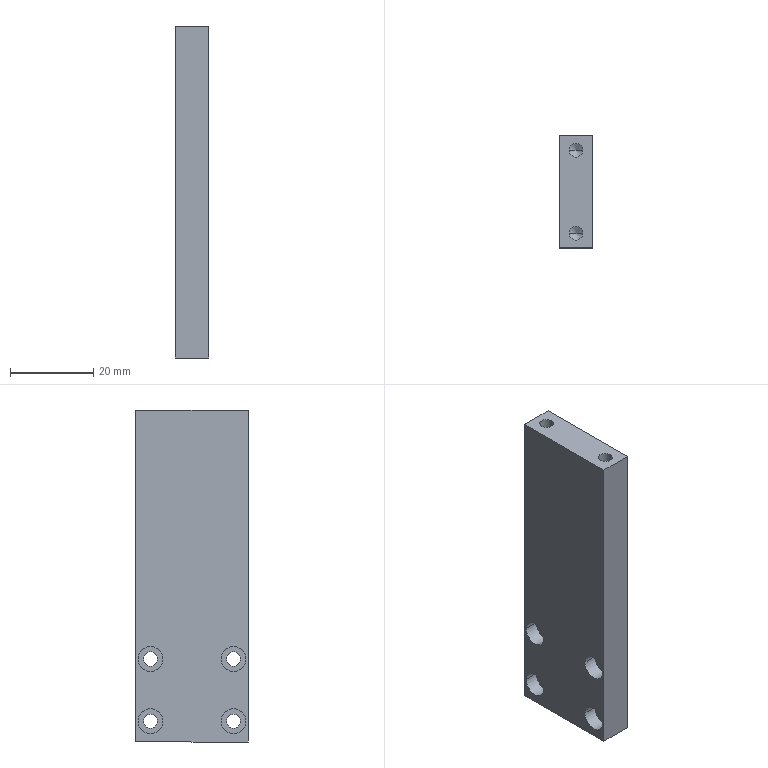Component | SolidWorks | JQ-2-0-004-2 | 1 solid | 34 faces | box 8 x 27 x 80 mm | volume 16526 mm3 | cylinder 20 | plane 10 | cone 4 | commonest cylinder face diameters 6 x8 3.4 x8 3.3 x4
build123d program:
from build123d import *

# Parameters (mm, degrees)
SKETCH1_W                                            = 27
SKETCH1_H                                            = 80
BOSS_EXTRUDE1_DEPTH                                  = 8
HOLE_SIZE_ACCORDING_TO_TYPE_1_OF_HEX_SOC_D           = 3.4
HOLE_SIZE_ACCORDING_TO_TYPE_1_OF_HEX_SOC_CBORE_D     = 6
HOLE_SIZE_ACCORDING_TO_TYPE_1_OF_HEX_SOC_CBORE_DEPTH = 3.4
M4_TAPPED_HOLE1_D                                    = 3.3
M4_TAPPED_HOLE1_DEPTH                                = 11.5
M4_TAPPED_HOLE1_TIP                                  = 0.9914


with BuildPart() as part:
    # Sketch1 → Boss-Extrude1 (new body)
    with BuildSketch(Plane.XY):
        with Locations((13.5, 40)):
            Rectangle(SKETCH1_W, SKETCH1_H)
    extrude(amount=BOSS_EXTRUDE1_DEPTH)

    # Hole Size according to type 1 of hex soc (through all)
    with Locations(Plane.XY.offset(8)):
        with Locations((3.5, 5), (23.5, 5), (3.5, 20), (23.5, 20)):
            CounterBoreHole(HOLE_SIZE_ACCORDING_TO_TYPE_1_OF_HEX_SOC_D / 2, HOLE_SIZE_ACCORDING_TO_TYPE_1_OF_HEX_SOC_CBORE_D / 2, HOLE_SIZE_ACCORDING_TO_TYPE_1_OF_HEX_SOC_CBORE_DEPTH)

    # M4 Tapped Hole1
    with Locations(Plane(origin=(0, 80, 0), x_dir=(-1, 0, 0), z_dir=(0, 1, 0))):
        with Locations((-23.5, 4), (-3.5, 4)):
            Hole(M4_TAPPED_HOLE1_D / 2, depth=M4_TAPPED_HOLE1_DEPTH)
            with Locations((0, 0, -(M4_TAPPED_HOLE1_DEPTH + M4_TAPPED_HOLE1_TIP / 2))):  # 118° drill point
                Cone(0, M4_TAPPED_HOLE1_D / 2, M4_TAPPED_HOLE1_TIP, mode=Mode.SUBTRACT)


solid = part.part

# Placed as in the assembly
solid = solid.moved(Location((-355.058, 42.839, 19.131), (90, -90, 0)))
STEP:
#1=COLOUR_RGB('',0.7922,0.8196,0.9333);
#2=FILL_AREA_STYLE_COLOUR('',#1);
#3=FILL_AREA_STYLE('',(#2));
#4=SURFACE_STYLE_FILL_AREA(#3);
#5=SURFACE_SIDE_STYLE('',(#4));
#6=SURFACE_STYLE_USAGE(.BOTH.,#5);
#7=PRESENTATION_STYLE_ASSIGNMENT((#6));
#8=CARTESIAN_POINT('',(-14.071,0.7614,3.45));
#9=VERTEX_POINT('',#8);
#10=CARTESIAN_POINT('',(-14.201,0.7614,3.45));
#11=VERTEX_POINT('',#10);
#12=CARTESIAN_POINT('',(-14.136,0.7614,3.45));
#13=DIRECTION('',(-0.,-0.,1.));
#14=DIRECTION('',(-1.,0.,0.));
#15=AXIS2_PLACEMENT_3D('',#12,#13,#14);
#16=CIRCLE('',#15,0.06496);
#17=EDGE_CURVE('',#9,#11,#16,.T.);
#18=ORIENTED_EDGE('',*,*,#17,.F.);
#19=CARTESIAN_POINT('',(-14.071,0.7614,3.903));
#20=VERTEX_POINT('',#19);
#21=CARTESIAN_POINT('',(-14.071,0.7614,3.903));
#22=DIRECTION('',(-0.,-0.,1.));
#23=VECTOR('',#22,39.37);
#24=LINE('',#21,#23);
#25=EDGE_CURVE('',#9,#20,#24,.T.);
#26=ORIENTED_EDGE('',*,*,#25,.T.);
#27=CARTESIAN_POINT('',(-14.201,0.7614,3.903));
#28=VERTEX_POINT('',#27);
#29=CARTESIAN_POINT('',(-14.136,0.7614,3.903));
#30=DIRECTION('',(-0.,-0.,1.));
#31=DIRECTION('',(-1.,0.,0.));
#32=AXIS2_PLACEMENT_3D('',#29,#30,#31);
#33=CIRCLE('',#32,0.06496);
#34=EDGE_CURVE('',#20,#28,#33,.T.);
#35=ORIENTED_EDGE('',*,*,#34,.T.);
#36=CARTESIAN_POINT('',(-14.201,0.7614,3.903));
#37=DIRECTION('',(-0.,-0.,1.));
#38=VECTOR('',#37,39.37);
#39=LINE('',#36,#38);
#40=EDGE_CURVE('',#11,#28,#39,.T.);
#41=ORIENTED_EDGE('',*,*,#40,.F.);
#42=EDGE_LOOP('',(#18,#26,#35,#41));
#43=FACE_OUTER_BOUND('',#42,.T.);
#44=CARTESIAN_POINT('',(-14.136,0.7614,3.903));
#45=DIRECTION('',(-0.,-0.,1.));
#46=DIRECTION('',(-1.,0.,0.));
#47=AXIS2_PLACEMENT_3D('',#44,#45,#46);
#48=CYLINDRICAL_SURFACE('',#47,0.06496);
#49=ADVANCED_FACE('',(#43),#48,.F.);
#50=CARTESIAN_POINT('',(-14.136,0.7614,3.411));
#51=VERTEX_POINT('',#50);
#52=CARTESIAN_POINT('',(-14.201,0.7614,3.45));
#53=DIRECTION('',(-0.8572,0.,0.515));
#54=VECTOR('',#53,39.37);
#55=LINE('',#52,#54);
#56=EDGE_CURVE('',#51,#11,#55,.T.);
#57=ORIENTED_EDGE('',*,*,#56,.F.);
#58=CARTESIAN_POINT('',(-14.071,0.7614,3.45));
#59=DIRECTION('',(0.8572,-0.,0.515));
#60=VECTOR('',#59,39.37);
#61=LINE('',#58,#60);
#62=EDGE_CURVE('',#51,#9,#61,.T.);
#63=ORIENTED_EDGE('',*,*,#62,.T.);
#64=ORIENTED_EDGE('',*,*,#17,.T.);
#65=EDGE_LOOP('',(#57,#63,#64));
#66=FACE_OUTER_BOUND('',#65,.T.);
#67=CARTESIAN_POINT('',(-14.136,0.7614,3.45));
#68=DIRECTION('',(-0.,-0.,1.));
#69=DIRECTION('',(-1.,0.,0.));
#70=AXIS2_PLACEMENT_3D('',#67,#68,#69);
#71=CONICAL_SURFACE('',#70,0.06496,1.03);
#72=ADVANCED_FACE('',(#66),#71,.F.);
#73=CARTESIAN_POINT('',(-14.071,1.549,3.45));
#74=VERTEX_POINT('',#73);
#75=CARTESIAN_POINT('',(-14.201,1.549,3.45));
#76=VERTEX_POINT('',#75);
#77=CARTESIAN_POINT('',(-14.136,1.549,3.45));
#78=DIRECTION('',(-0.,-0.,1.));
#79=DIRECTION('',(-1.,0.,0.));
#80=AXIS2_PLACEMENT_3D('',#77,#78,#79);
#81=CIRCLE('',#80,0.06496);
#82=EDGE_CURVE('',#74,#76,#81,.T.);
#83=ORIENTED_EDGE('',*,*,#82,.F.);
#84=CARTESIAN_POINT('',(-14.071,1.549,3.903));
#85=VERTEX_POINT('',#84);
#86=CARTESIAN_POINT('',(-14.071,1.549,3.903));
#87=DIRECTION('',(-0.,-0.,1.));
#88=VECTOR('',#87,39.37);
#89=LINE('',#86,#88);
#90=EDGE_CURVE('',#74,#85,#89,.T.);
#91=ORIENTED_EDGE('',*,*,#90,.T.);
#92=CARTESIAN_POINT('',(-14.201,1.549,3.903));
#93=VERTEX_POINT('',#92);
#94=CARTESIAN_POINT('',(-14.136,1.549,3.903));
#95=DIRECTION('',(-0.,-0.,1.));
#96=DIRECTION('',(-1.,0.,0.));
#97=AXIS2_PLACEMENT_3D('',#94,#95,#96);
#98=CIRCLE('',#97,0.06496);
#99=EDGE_CURVE('',#85,#93,#98,.T.);
#100=ORIENTED_EDGE('',*,*,#99,.T.);
#101=CARTESIAN_POINT('',(-14.201,1.549,3.903));
#102=DIRECTION('',(-0.,-0.,1.));
#103=VECTOR('',#102,39.37);
#104=LINE('',#101,#103);
#105=EDGE_CURVE('',#76,#93,#104,.T.);
#106=ORIENTED_EDGE('',*,*,#105,.F.);
#107=EDGE_LOOP('',(#83,#91,#100,#106));
#108=FACE_OUTER_BOUND('',#107,.T.);
#109=CARTESIAN_POINT('',(-14.136,1.549,3.903));
#110=DIRECTION('',(-0.,-0.,1.));
#111=DIRECTION('',(-1.,0.,0.));
#112=AXIS2_PLACEMENT_3D('',#109,#110,#111);
#113=CYLINDRICAL_SURFACE('',#112,0.06496);
#114=ADVANCED_FACE('',(#108),#113,.F.);
#115=CARTESIAN_POINT('',(-14.136,1.549,3.411));
#116=VERTEX_POINT('',#115);
#117=CARTESIAN_POINT('',(-14.201,1.549,3.45));
#118=DIRECTION('',(-0.8572,0.,0.515));
#119=VECTOR('',#118,39.37);
#120=LINE('',#117,#119);
#121=EDGE_CURVE('',#116,#76,#120,.T.);
#122=ORIENTED_EDGE('',*,*,#121,.F.);
#123=CARTESIAN_POINT('',(-14.071,1.549,3.45));
#124=DIRECTION('',(0.8572,-0.,0.515));
#125=VECTOR('',#124,39.37);
#126=LINE('',#123,#125);
#127=EDGE_CURVE('',#116,#74,#126,.T.);
#128=ORIENTED_EDGE('',*,*,#127,.T.);
#129=ORIENTED_EDGE('',*,*,#82,.T.);
#130=EDGE_LOOP('',(#122,#128,#129));
#131=FACE_OUTER_BOUND('',#130,.T.);
#132=CARTESIAN_POINT('',(-14.136,1.549,3.45));
#133=DIRECTION('',(-0.,-0.,1.));
#134=DIRECTION('',(-1.,0.,0.));
#135=AXIS2_PLACEMENT_3D('',#132,#133,#134);
#136=CONICAL_SURFACE('',#135,0.06496,1.03);
#137=ADVANCED_FACE('',(#131),#136,.F.);
#138=CARTESIAN_POINT('',(-14.16,1.667,0.95));
#139=VERTEX_POINT('',#138);
#140=CARTESIAN_POINT('',(-14.16,1.431,0.95));
#141=VERTEX_POINT('',#140);
#142=CARTESIAN_POINT('',(-14.16,1.549,0.95));
#143=DIRECTION('',(-1.,0.,-0.));
#144=DIRECTION('',(0.,-1.,0.));
#145=AXIS2_PLACEMENT_3D('',#142,#143,#144);
#146=CIRCLE('',#145,0.1181);
#147=EDGE_CURVE('',#139,#141,#146,.T.);
#148=ORIENTED_EDGE('',*,*,#147,.F.);
#149=CARTESIAN_POINT('',(-14.294,1.667,0.95));
#150=VERTEX_POINT('',#149);
#151=CARTESIAN_POINT('',(-14.294,1.667,0.95));
#152=DIRECTION('',(-1.,0.,-0.));
#153=VECTOR('',#152,39.37);
#154=LINE('',#151,#153);
#155=EDGE_CURVE('',#139,#150,#154,.T.);
#156=ORIENTED_EDGE('',*,*,#155,.T.);
#157=CARTESIAN_POINT('',(-14.294,1.431,0.95));
#158=VERTEX_POINT('',#157);
#159=CARTESIAN_POINT('',(-14.294,1.549,0.95));
#160=DIRECTION('',(-1.,0.,-0.));
#161=DIRECTION('',(0.,-1.,0.));
#162=AXIS2_PLACEMENT_3D('',#159,#160,#161);
#163=CIRCLE('',#162,0.1181);
#164=EDGE_CURVE('',#150,#158,#163,.T.);
#165=ORIENTED_EDGE('',*,*,#164,.T.);
#166=CARTESIAN_POINT('',(-14.294,1.431,0.95));
#167=DIRECTION('',(-1.,0.,-0.));
#168=VECTOR('',#167,39.37);
#169=LINE('',#166,#168);
#170=EDGE_CURVE('',#141,#158,#169,.T.);
#171=ORIENTED_EDGE('',*,*,#170,.F.);
#172=EDGE_LOOP('',(#148,#156,#165,#171));
#173=FACE_OUTER_BOUND('',#172,.T.);
#174=CARTESIAN_POINT('',(-14.294,1.549,0.95));
#175=DIRECTION('',(-1.,0.,-0.));
#176=DIRECTION('',(0.,-1.,0.));
#177=AXIS2_PLACEMENT_3D('',#174,#175,#176);
#178=CYLINDRICAL_SURFACE('',#177,0.1181);
#179=ADVANCED_FACE('',(#173),#178,.F.);
#180=CARTESIAN_POINT('',(-13.979,1.616,0.95));
#181=VERTEX_POINT('',#180);
#182=CARTESIAN_POINT('',(-13.979,1.482,0.95));
#183=VERTEX_POINT('',#182);
#184=CARTESIAN_POINT('',(-13.979,1.549,0.95));
#185=DIRECTION('',(-1.,0.,-0.));
#186=DIRECTION('',(0.,-1.,0.));
#187=AXIS2_PLACEMENT_3D('',#184,#185,#186);
#188=CIRCLE('',#187,0.06693);
#189=EDGE_CURVE('',#181,#183,#188,.T.);
#190=ORIENTED_EDGE('',*,*,#189,.F.);
#191=CARTESIAN_POINT('',(-14.16,1.616,0.95));
#192=VERTEX_POINT('',#191);
#193=CARTESIAN_POINT('',(-14.294,1.616,0.95));
#194=DIRECTION('',(-1.,0.,-0.));
#195=VECTOR('',#194,39.37);
#196=LINE('',#193,#195);
#197=EDGE_CURVE('',#181,#192,#196,.T.);
#198=ORIENTED_EDGE('',*,*,#197,.T.);
#199=CARTESIAN_POINT('',(-14.16,1.482,0.95));
#200=VERTEX_POINT('',#199);
#201=CARTESIAN_POINT('',(-14.16,1.549,0.95));
#202=DIRECTION('',(-1.,0.,-0.));
#203=DIRECTION('',(0.,-1.,0.));
#204=AXIS2_PLACEMENT_3D('',#201,#202,#203);
#205=CIRCLE('',#204,0.06693);
#206=EDGE_CURVE('',#192,#200,#205,.T.);
#207=ORIENTED_EDGE('',*,*,#206,.T.);
#208=CARTESIAN_POINT('',(-14.294,1.482,0.95));
#209=DIRECTION('',(-1.,0.,-0.));
#210=VECTOR('',#209,39.37);
#211=LINE('',#208,#210);
#212=EDGE_CURVE('',#183,#200,#211,.T.);
#213=ORIENTED_EDGE('',*,*,#212,.F.);
#214=EDGE_LOOP('',(#190,#198,#207,#213));
#215=FACE_OUTER_BOUND('',#214,.T.);
#216=CARTESIAN_POINT('',(-14.294,1.549,0.95));
#217=DIRECTION('',(-1.,0.,-0.));
#218=DIRECTION('',(0.,-1.,0.));
#219=AXIS2_PLACEMENT_3D('',#216,#217,#218);
#220=CYLINDRICAL_SURFACE('',#219,0.06693);
#221=ADVANCED_FACE('',(#215),#220,.F.);
#222=CARTESIAN_POINT('',(-14.16,0.8795,0.95));
#223=VERTEX_POINT('',#222);
#224=CARTESIAN_POINT('',(-14.16,0.6433,0.95));
#225=VERTEX_POINT('',#224);
#226=CARTESIAN_POINT('',(-14.16,0.7614,0.95));
#227=DIRECTION('',(-1.,0.,-0.));
#228=DIRECTION('',(0.,-1.,0.));
#229=AXIS2_PLACEMENT_3D('',#226,#227,#228);
#230=CIRCLE('',#229,0.1181);
#231=EDGE_CURVE('',#223,#225,#230,.T.);
#232=ORIENTED_EDGE('',*,*,#231,.F.);
#233=CARTESIAN_POINT('',(-14.294,0.8795,0.95));
#234=VERTEX_POINT('',#233);
#235=CARTESIAN_POINT('',(-14.294,0.8795,0.95));
#236=DIRECTION('',(-1.,0.,-0.));
#237=VECTOR('',#236,39.37);
#238=LINE('',#235,#237);
#239=EDGE_CURVE('',#223,#234,#238,.T.);
#240=ORIENTED_EDGE('',*,*,#239,.T.);
#241=CARTESIAN_POINT('',(-14.294,0.6433,0.95));
#242=VERTEX_POINT('',#241);
#243=CARTESIAN_POINT('',(-14.294,0.7614,0.95));
#244=DIRECTION('',(-1.,0.,-0.));
#245=DIRECTION('',(0.,-1.,0.));
#246=AXIS2_PLACEMENT_3D('',#243,#244,#245);
#247=CIRCLE('',#246,0.1181);
#248=EDGE_CURVE('',#234,#242,#247,.T.);
#249=ORIENTED_EDGE('',*,*,#248,.T.);
#250=CARTESIAN_POINT('',(-14.294,0.6433,0.95));
#251=DIRECTION('',(-1.,0.,-0.));
#252=VECTOR('',#251,39.37);
#253=LINE('',#250,#252);
#254=EDGE_CURVE('',#225,#242,#253,.T.);
#255=ORIENTED_EDGE('',*,*,#254,.F.);
#256=EDGE_LOOP('',(#232,#240,#249,#255));
#257=FACE_OUTER_BOUND('',#256,.T.);
#258=CARTESIAN_POINT('',(-14.294,0.7614,0.95));
#259=DIRECTION('',(-1.,0.,-0.));
#260=DIRECTION('',(0.,-1.,0.));
#261=AXIS2_PLACEMENT_3D('',#258,#259,#260);
#262=CYLINDRICAL_SURFACE('',#261,0.1181);
#263=ADVANCED_FACE('',(#257),#262,.F.);
#264=CARTESIAN_POINT('',(-13.979,0.8283,0.95));
#265=VERTEX_POINT('',#264);
#266=CARTESIAN_POINT('',(-13.979,0.6945,0.95));
#267=VERTEX_POINT('',#266);
#268=CARTESIAN_POINT('',(-13.979,0.7614,0.95));
#269=DIRECTION('',(-1.,0.,-0.));
#270=DIRECTION('',(0.,-1.,0.));
#271=AXIS2_PLACEMENT_3D('',#268,#269,#270);
#272=CIRCLE('',#271,0.06693);
#273=EDGE_CURVE('',#265,#267,#272,.T.);
#274=ORIENTED_EDGE('',*,*,#273,.F.);
#275=CARTESIAN_POINT('',(-14.16,0.8283,0.95));
#276=VERTEX_POINT('',#275);
#277=CARTESIAN_POINT('',(-14.294,0.8283,0.95));
#278=DIRECTION('',(-1.,0.,-0.));
#279=VECTOR('',#278,39.37);
#280=LINE('',#277,#279);
#281=EDGE_CURVE('',#265,#276,#280,.T.);
#282=ORIENTED_EDGE('',*,*,#281,.T.);
#283=CARTESIAN_POINT('',(-14.16,0.6945,0.95));
#284=VERTEX_POINT('',#283);
#285=CARTESIAN_POINT('',(-14.16,0.7614,0.95));
#286=DIRECTION('',(-1.,0.,-0.));
#287=DIRECTION('',(0.,-1.,0.));
#288=AXIS2_PLACEMENT_3D('',#285,#286,#287);
#289=CIRCLE('',#288,0.06693);
#290=EDGE_CURVE('',#276,#284,#289,.T.);
#291=ORIENTED_EDGE('',*,*,#290,.T.);
#292=CARTESIAN_POINT('',(-14.294,0.6945,0.95));
#293=DIRECTION('',(-1.,0.,-0.));
#294=VECTOR('',#293,39.37);
#295=LINE('',#292,#294);
#296=EDGE_CURVE('',#267,#284,#295,.T.);
#297=ORIENTED_EDGE('',*,*,#296,.F.);
#298=EDGE_LOOP('',(#274,#282,#291,#297));
#299=FACE_OUTER_BOUND('',#298,.T.);
#300=CARTESIAN_POINT('',(-14.294,0.7614,0.95));
#301=DIRECTION('',(-1.,0.,-0.));
#302=DIRECTION('',(0.,-1.,0.));
#303=AXIS2_PLACEMENT_3D('',#300,#301,#302);
#304=CYLINDRICAL_SURFACE('',#303,0.06693);
#305=ADVANCED_FACE('',(#299),#304,.F.);
#306=CARTESIAN_POINT('',(-14.16,1.667,1.541));
#307=VERTEX_POINT('',#306);
#308=CARTESIAN_POINT('',(-14.16,1.431,1.541));
#309=VERTEX_POINT('',#308);
#310=CARTESIAN_POINT('',(-14.16,1.549,1.541));
#311=DIRECTION('',(-1.,0.,-0.));
#312=DIRECTION('',(0.,-1.,0.));
#313=AXIS2_PLACEMENT_3D('',#310,#311,#312);
#314=CIRCLE('',#313,0.1181);
#315=EDGE_CURVE('',#307,#309,#314,.T.);
#316=ORIENTED_EDGE('',*,*,#315,.F.);
#317=CARTESIAN_POINT('',(-14.294,1.667,1.541));
#318=VERTEX_POINT('',#317);
#319=CARTESIAN_POINT('',(-14.294,1.667,1.541));
#320=DIRECTION('',(-1.,0.,-0.));
#321=VECTOR('',#320,39.37);
#322=LINE('',#319,#321);
#323=EDGE_CURVE('',#307,#318,#322,.T.);
#324=ORIENTED_EDGE('',*,*,#323,.T.);
#325=CARTESIAN_POINT('',(-14.294,1.431,1.541));
#326=VERTEX_POINT('',#325);
#327=CARTESIAN_POINT('',(-14.294,1.549,1.541));
#328=DIRECTION('',(-1.,0.,-0.));
#329=DIRECTION('',(0.,-1.,0.));
#330=AXIS2_PLACEMENT_3D('',#327,#328,#329);
#331=CIRCLE('',#330,0.1181);
#332=EDGE_CURVE('',#318,#326,#331,.T.);
#333=ORIENTED_EDGE('',*,*,#332,.T.);
#334=CARTESIAN_POINT('',(-14.294,1.431,1.541));
#335=DIRECTION('',(-1.,0.,-0.));
#336=VECTOR('',#335,39.37);
#337=LINE('',#334,#336);
#338=EDGE_CURVE('',#309,#326,#337,.T.);
#339=ORIENTED_EDGE('',*,*,#338,.F.);
#340=EDGE_LOOP('',(#316,#324,#333,#339));
#341=FACE_OUTER_BOUND('',#340,.T.);
#342=CARTESIAN_POINT('',(-14.294,1.549,1.541));
#343=DIRECTION('',(-1.,0.,-0.));
#344=DIRECTION('',(0.,-1.,0.));
#345=AXIS2_PLACEMENT_3D('',#342,#343,#344);
#346=CYLINDRICAL_SURFACE('',#345,0.1181);
#347=ADVANCED_FACE('',(#341),#346,.F.);
#348=CARTESIAN_POINT('',(-13.979,1.616,1.541));
#349=VERTEX_POINT('',#348);
#350=CARTESIAN_POINT('',(-13.979,1.482,1.541));
#351=VERTEX_POINT('',#350);
#352=CARTESIAN_POINT('',(-13.979,1.549,1.541));
#353=DIRECTION('',(-1.,0.,-0.));
#354=DIRECTION('',(0.,-1.,0.));
#355=AXIS2_PLACEMENT_3D('',#352,#353,#354);
#356=CIRCLE('',#355,0.06693);
#357=EDGE_CURVE('',#349,#351,#356,.T.);
#358=ORIENTED_EDGE('',*,*,#357,.F.);
#359=CARTESIAN_POINT('',(-14.16,1.616,1.541));
#360=VERTEX_POINT('',#359);
#361=CARTESIAN_POINT('',(-14.294,1.616,1.541));
#362=DIRECTION('',(-1.,0.,-0.));
#363=VECTOR('',#362,39.37);
#364=LINE('',#361,#363);
#365=EDGE_CURVE('',#349,#360,#364,.T.);
#366=ORIENTED_EDGE('',*,*,#365,.T.);
#367=CARTESIAN_POINT('',(-14.16,1.482,1.541));
#368=VERTEX_POINT('',#367);
#369=CARTESIAN_POINT('',(-14.16,1.549,1.541));
#370=DIRECTION('',(-1.,0.,-0.));
#371=DIRECTION('',(0.,-1.,0.));
#372=AXIS2_PLACEMENT_3D('',#369,#370,#371);
#373=CIRCLE('',#372,0.06693);
#374=EDGE_CURVE('',#360,#368,#373,.T.);
#375=ORIENTED_EDGE('',*,*,#374,.T.);
#376=CARTESIAN_POINT('',(-14.294,1.482,1.541));
#377=DIRECTION('',(-1.,0.,-0.));
#378=VECTOR('',#377,39.37);
#379=LINE('',#376,#378);
#380=EDGE_CURVE('',#351,#368,#379,.T.);
#381=ORIENTED_EDGE('',*,*,#380,.F.);
#382=EDGE_LOOP('',(#358,#366,#375,#381));
#383=FACE_OUTER_BOUND('',#382,.T.);
#384=CARTESIAN_POINT('',(-14.294,1.549,1.541));
#385=DIRECTION('',(-1.,0.,-0.));
#386=DIRECTION('',(0.,-1.,0.));
#387=AXIS2_PLACEMENT_3D('',#384,#385,#386);
#388=CYLINDRICAL_SURFACE('',#387,0.06693);
#389=ADVANCED_FACE('',(#383),#388,.F.);
#390=CARTESIAN_POINT('',(-14.16,0.8795,1.541));
#391=VERTEX_POINT('',#390);
#392=CARTESIAN_POINT('',(-14.16,0.6433,1.541));
#393=VERTEX_POINT('',#392);
#394=CARTESIAN_POINT('',(-14.16,0.7614,1.541));
#395=DIRECTION('',(-1.,0.,-0.));
#396=DIRECTION('',(0.,-1.,0.));
#397=AXIS2_PLACEMENT_3D('',#394,#395,#396);
#398=CIRCLE('',#397,0.1181);
#399=EDGE_CURVE('',#391,#393,#398,.T.);
#400=ORIENTED_EDGE('',*,*,#399,.F.);
#401=CARTESIAN_POINT('',(-14.294,0.8795,1.541));
#402=VERTEX_POINT('',#401);
#403=CARTESIAN_POINT('',(-14.294,0.8795,1.541));
#404=DIRECTION('',(-1.,0.,-0.));
#405=VECTOR('',#404,39.37);
#406=LINE('',#403,#405);
#407=EDGE_CURVE('',#391,#402,#406,.T.);
#408=ORIENTED_EDGE('',*,*,#407,.T.);
#409=CARTESIAN_POINT('',(-14.294,0.6433,1.541));
#410=VERTEX_POINT('',#409);
#411=CARTESIAN_POINT('',(-14.294,0.7614,1.541));
#412=DIRECTION('',(-1.,0.,-0.));
#413=DIRECTION('',(0.,-1.,0.));
#414=AXIS2_PLACEMENT_3D('',#411,#412,#413);
#415=CIRCLE('',#414,0.1181);
#416=EDGE_CURVE('',#402,#410,#415,.T.);
#417=ORIENTED_EDGE('',*,*,#416,.T.);
#418=CARTESIAN_POINT('',(-14.294,0.6433,1.541));
#419=DIRECTION('',(-1.,0.,-0.));
#420=VECTOR('',#419,39.37);
#421=LINE('',#418,#420);
#422=EDGE_CURVE('',#393,#410,#421,.T.);
#423=ORIENTED_EDGE('',*,*,#422,.F.);
#424=EDGE_LOOP('',(#400,#408,#417,#423));
#425=FACE_OUTER_BOUND('',#424,.T.);
#426=CARTESIAN_POINT('',(-14.294,0.7614,1.541));
#427=DIRECTION('',(-1.,0.,-0.));
#428=DIRECTION('',(0.,-1.,0.));
#429=AXIS2_PLACEMENT_3D('',#426,#427,#428);
#430=CYLINDRICAL_SURFACE('',#429,0.1181);
#431=ADVANCED_FACE('',(#425),#430,.F.);
#432=CARTESIAN_POINT('',(-13.979,0.8283,1.541));
#433=VERTEX_POINT('',#432);
#434=CARTESIAN_POINT('',(-13.979,0.6945,1.541));
#435=VERTEX_POINT('',#434);
#436=CARTESIAN_POINT('',(-13.979,0.7614,1.541));
#437=DIRECTION('',(-1.,0.,-0.));
#438=DIRECTION('',(0.,-1.,0.));
#439=AXIS2_PLACEMENT_3D('',#436,#437,#438);
#440=CIRCLE('',#439,0.06693);
#441=EDGE_CURVE('',#433,#435,#440,.T.);
#442=ORIENTED_EDGE('',*,*,#441,.F.);
#443=CARTESIAN_POINT('',(-14.16,0.8283,1.541));
#444=VERTEX_POINT('',#443);
#445=CARTESIAN_POINT('',(-14.294,0.8283,1.541));
#446=DIRECTION('',(-1.,0.,-0.));
#447=VECTOR('',#446,39.37);
#448=LINE('',#445,#447);
#449=EDGE_CURVE('',#433,#444,#448,.T.);
#450=ORIENTED_EDGE('',*,*,#449,.T.);
#451=CARTESIAN_POINT('',(-14.16,0.6945,1.541));
#452=VERTEX_POINT('',#451);
#453=CARTESIAN_POINT('',(-14.16,0.7614,1.541));
#454=DIRECTION('',(-1.,0.,-0.));
#455=DIRECTION('',(0.,-1.,0.));
#456=AXIS2_PLACEMENT_3D('',#453,#454,#455);
#457=CIRCLE('',#456,0.06693);
#458=EDGE_CURVE('',#444,#452,#457,.T.);
#459=ORIENTED_EDGE('',*,*,#458,.T.);
#460=CARTESIAN_POINT('',(-14.294,0.6945,1.541));
#461=DIRECTION('',(-1.,0.,-0.));
#462=VECTOR('',#461,39.37);
#463=LINE('',#460,#462);
#464=EDGE_CURVE('',#435,#452,#463,.T.);
#465=ORIENTED_EDGE('',*,*,#464,.F.);
#466=EDGE_LOOP('',(#442,#450,#459,#465));
#467=FACE_OUTER_BOUND('',#466,.T.);
#468=CARTESIAN_POINT('',(-14.294,0.7614,1.541));
#469=DIRECTION('',(-1.,0.,-0.));
#470=DIRECTION('',(0.,-1.,0.));
#471=AXIS2_PLACEMENT_3D('',#468,#469,#470);
#472=CYLINDRICAL_SURFACE('',#471,0.06693);
#473=ADVANCED_FACE('',(#467),#472,.F.);
#474=CARTESIAN_POINT('',(-14.294,0.7614,0.95));
#475=DIRECTION('',(-1.,0.,-0.));
#476=DIRECTION('',(0.,-1.,0.));
#477=AXIS2_PLACEMENT_3D('',#474,#475,#476);
#478=CIRCLE('',#477,0.1181);
#479=EDGE_CURVE('',#242,#234,#478,.T.);
#480=ORIENTED_EDGE('',*,*,#479,.F.);
#481=ORIENTED_EDGE('',*,*,#248,.F.);
#482=EDGE_LOOP('',(#480,#481));
#483=FACE_BOUND('',#482,.T.);
#484=CARTESIAN_POINT('',(-14.294,1.549,1.541));
#485=DIRECTION('',(-1.,0.,-0.));
#486=DIRECTION('',(0.,-1.,0.));
#487=AXIS2_PLACEMENT_3D('',#484,#485,#486);
#488=CIRCLE('',#487,0.1181);
#489=EDGE_CURVE('',#326,#318,#488,.T.);
#490=ORIENTED_EDGE('',*,*,#489,.F.);
#491=ORIENTED_EDGE('',*,*,#332,.F.);
#492=EDGE_LOOP('',(#490,#491));
#493=FACE_BOUND('',#492,.T.);
#494=CARTESIAN_POINT('',(-14.294,0.7614,1.541));
#495=DIRECTION('',(-1.,0.,-0.));
#496=DIRECTION('',(0.,-1.,0.));
#497=AXIS2_PLACEMENT_3D('',#494,#495,#496);
#498=CIRCLE('',#497,0.1181);
#499=EDGE_CURVE('',#410,#402,#498,.T.);
#500=ORIENTED_EDGE('',*,*,#499,.F.);
#501=ORIENTED_EDGE('',*,*,#416,.F.);
#502=EDGE_LOOP('',(#500,#501));
#503=FACE_BOUND('',#502,.T.);
#504=CARTESIAN_POINT('',(-14.294,1.687,3.903));
#505=VERTEX_POINT('',#504);
#506=CARTESIAN_POINT('',(-14.294,1.687,0.7532));
#507=VERTEX_POINT('',#506);
#508=CARTESIAN_POINT('',(-14.294,1.687,0.7532));
#509=DIRECTION('',(0.,0.,-1.));
#510=VECTOR('',#509,39.37);
#511=LINE('',#508,#510);
#512=EDGE_CURVE('',#505,#507,#511,.T.);
#513=ORIENTED_EDGE('',*,*,#512,.T.);
#514=CARTESIAN_POINT('',(-14.294,0.6236,0.7532));
#515=VERTEX_POINT('',#514);
#516=CARTESIAN_POINT('',(-14.294,1.687,0.7532));
#517=DIRECTION('',(-0.,-1.,-0.));
#518=VECTOR('',#517,39.37);
#519=LINE('',#516,#518);
#520=EDGE_CURVE('',#507,#515,#519,.T.);
#521=ORIENTED_EDGE('',*,*,#520,.T.);
#522=CARTESIAN_POINT('',(-14.294,0.6236,3.903));
#523=VERTEX_POINT('',#522);
#524=CARTESIAN_POINT('',(-14.294,0.6236,0.7532));
#525=DIRECTION('',(-0.,-0.,1.));
#526=VECTOR('',#525,39.37);
#527=LINE('',#524,#526);
#528=EDGE_CURVE('',#515,#523,#527,.T.);
#529=ORIENTED_EDGE('',*,*,#528,.T.);
#530=CARTESIAN_POINT('',(-14.294,1.687,3.903));
#531=DIRECTION('',(0.,1.,0.));
#532=VECTOR('',#531,39.37);
#533=LINE('',#530,#532);
#534=EDGE_CURVE('',#523,#505,#533,.T.);
#535=ORIENTED_EDGE('',*,*,#534,.T.);
#536=EDGE_LOOP('',(#513,#521,#529,#535));
#537=FACE_OUTER_BOUND('',#536,.T.);
#538=CARTESIAN_POINT('',(-14.294,1.549,0.95));
#539=DIRECTION('',(-1.,0.,-0.));
#540=DIRECTION('',(0.,-1.,0.));
#541=AXIS2_PLACEMENT_3D('',#538,#539,#540);
#542=CIRCLE('',#541,0.1181);
#543=EDGE_CURVE('',#158,#150,#542,.T.);
#544=ORIENTED_EDGE('',*,*,#543,.F.);
#545=ORIENTED_EDGE('',*,*,#164,.F.);
#546=EDGE_LOOP('',(#544,#545));
#547=FACE_BOUND('',#546,.T.);
#548=CARTESIAN_POINT('',(-14.294,1.687,3.903));
#549=DIRECTION('',(1.,-0.,0.));
#550=DIRECTION('',(0.,1.,0.));
#551=AXIS2_PLACEMENT_3D('',#548,#549,#550);
#552=PLANE('',#551);
#553=ADVANCED_FACE('',(#483,#493,#503,#537,#547),#552,.F.);
#554=CARTESIAN_POINT('',(-13.979,1.687,3.903));
#555=VERTEX_POINT('',#554);
#556=CARTESIAN_POINT('',(-13.979,1.687,0.7532));
#557=VERTEX_POINT('',#556);
#558=CARTESIAN_POINT('',(-13.979,1.687,0.7532));
#559=DIRECTION('',(0.,0.,-1.));
#560=VECTOR('',#559,39.37);
#561=LINE('',#558,#560);
#562=EDGE_CURVE('',#555,#557,#561,.T.);
#563=ORIENTED_EDGE('',*,*,#562,.T.);
#564=CARTESIAN_POINT('',(-14.294,1.687,0.7532));
#565=DIRECTION('',(1.,-0.,0.));
#566=VECTOR('',#565,39.37);
#567=LINE('',#564,#566);
#568=EDGE_CURVE('',#507,#557,#567,.T.);
#569=ORIENTED_EDGE('',*,*,#568,.F.);
#570=ORIENTED_EDGE('',*,*,#512,.F.);
#571=CARTESIAN_POINT('',(-14.294,1.687,3.903));
#572=DIRECTION('',(1.,-0.,0.));
#573=VECTOR('',#572,39.37);
#574=LINE('',#571,#573);
#575=EDGE_CURVE('',#505,#555,#574,.T.);
#576=ORIENTED_EDGE('',*,*,#575,.T.);
#577=EDGE_LOOP('',(#563,#569,#570,#576));
#578=FACE_OUTER_BOUND('',#577,.T.);
#579=CARTESIAN_POINT('',(-14.294,1.687,0.7532));
#580=DIRECTION('',(-0.,-1.,-0.));
#581=DIRECTION('',(1.,-0.,0.));
#582=AXIS2_PLACEMENT_3D('',#579,#580,#581);
#583=PLANE('',#582);
#584=ADVANCED_FACE('',(#578),#583,.F.);
#585=CARTESIAN_POINT('',(-13.979,0.6236,0.7532));
#586=VERTEX_POINT('',#585);
#587=CARTESIAN_POINT('',(-13.979,1.687,0.7532));
#588=DIRECTION('',(-0.,-1.,-0.));
#589=VECTOR('',#588,39.37);
#590=LINE('',#587,#589);
#591=EDGE_CURVE('',#557,#586,#590,.T.);
#592=ORIENTED_EDGE('',*,*,#591,.T.);
#593=CARTESIAN_POINT('',(-14.294,0.6236,0.7532));
#594=DIRECTION('',(1.,-0.,0.));
#595=VECTOR('',#594,39.37);
#596=LINE('',#593,#595);
#597=EDGE_CURVE('',#515,#586,#596,.T.);
#598=ORIENTED_EDGE('',*,*,#597,.F.);
#599=ORIENTED_EDGE('',*,*,#520,.F.);
#600=ORIENTED_EDGE('',*,*,#568,.T.);
#601=EDGE_LOOP('',(#592,#598,#599,#600));
#602=FACE_OUTER_BOUND('',#601,.T.);
#603=CARTESIAN_POINT('',(-14.294,1.687,0.7532));
#604=DIRECTION('',(-0.,-0.,1.));
#605=DIRECTION('',(-1.,0.,-0.));
#606=AXIS2_PLACEMENT_3D('',#603,#604,#605);
#607=PLANE('',#606);
#608=ADVANCED_FACE('',(#602),#607,.F.);
#609=CARTESIAN_POINT('',(-13.979,0.6236,3.903));
#610=VERTEX_POINT('',#609);
#611=CARTESIAN_POINT('',(-13.979,0.6236,0.7532));
#612=DIRECTION('',(-0.,-0.,1.));
#613=VECTOR('',#612,39.37);
#614=LINE('',#611,#613);
#615=EDGE_CURVE('',#586,#610,#614,.T.);
#616=ORIENTED_EDGE('',*,*,#615,.T.);
#617=CARTESIAN_POINT('',(-14.294,0.6236,3.903));
#618=DIRECTION('',(1.,-0.,0.));
#619=VECTOR('',#618,39.37);
#620=LINE('',#617,#619);
#621=EDGE_CURVE('',#523,#610,#620,.T.);
#622=ORIENTED_EDGE('',*,*,#621,.F.);
#623=ORIENTED_EDGE('',*,*,#528,.F.);
#624=ORIENTED_EDGE('',*,*,#597,.T.);
#625=EDGE_LOOP('',(#616,#622,#623,#624));
#626=FACE_OUTER_BOUND('',#625,.T.);
#627=CARTESIAN_POINT('',(-14.294,0.6236,0.7532));
#628=DIRECTION('',(0.,1.,0.));
#629=DIRECTION('',(-1.,0.,-0.));
#630=AXIS2_PLACEMENT_3D('',#627,#628,#629);
#631=PLANE('',#630);
#632=ADVANCED_FACE('',(#626),#631,.F.);
#633=CARTESIAN_POINT('',(-14.136,0.7614,3.903));
#634=DIRECTION('',(-0.,-0.,1.));
#635=DIRECTION('',(-1.,0.,0.));
#636=AXIS2_PLACEMENT_3D('',#633,#634,#635);
#637=CIRCLE('',#636,0.06496);
#638=EDGE_CURVE('',#28,#20,#637,.T.);
#639=ORIENTED_EDGE('',*,*,#638,.F.);
#640=ORIENTED_EDGE('',*,*,#34,.F.);
#641=EDGE_LOOP('',(#639,#640));
#642=FACE_BOUND('',#641,.T.);
#643=CARTESIAN_POINT('',(-14.136,1.549,3.903));
#644=DIRECTION('',(-0.,-0.,1.));
#645=DIRECTION('',(-1.,0.,0.));
#646=AXIS2_PLACEMENT_3D('',#643,#644,#645);
#647=CIRCLE('',#646,0.06496);
#648=EDGE_CURVE('',#93,#85,#647,.T.);
#649=ORIENTED_EDGE('',*,*,#648,.F.);
#650=ORIENTED_EDGE('',*,*,#99,.F.);
#651=EDGE_LOOP('',(#649,#650));
#652=FACE_BOUND('',#651,.T.);
#653=CARTESIAN_POINT('',(-13.979,1.687,3.903));
#654=DIRECTION('',(0.,1.,0.));
#655=VECTOR('',#654,39.37);
#656=LINE('',#653,#655);
#657=EDGE_CURVE('',#610,#555,#656,.T.);
#658=ORIENTED_EDGE('',*,*,#657,.T.);
#659=ORIENTED_EDGE('',*,*,#575,.F.);
#660=ORIENTED_EDGE('',*,*,#534,.F.);
#661=ORIENTED_EDGE('',*,*,#621,.T.);
#662=EDGE_LOOP('',(#658,#659,#660,#661));
#663=FACE_OUTER_BOUND('',#662,.T.);
#664=CARTESIAN_POINT('',(-14.294,1.687,3.903));
#665=DIRECTION('',(0.,0.,-1.));
#666=DIRECTION('',(1.,-0.,0.));
#667=AXIS2_PLACEMENT_3D('',#664,#665,#666);
#668=PLANE('',#667);
#669=ADVANCED_FACE('',(#642,#652,#663),#668,.F.);
#670=CARTESIAN_POINT('',(-13.979,1.549,0.95));
#671=DIRECTION('',(-1.,0.,-0.));
#672=DIRECTION('',(0.,-1.,0.));
#673=AXIS2_PLACEMENT_3D('',#670,#671,#672);
#674=CIRCLE('',#673,0.06693);
#675=EDGE_CURVE('',#183,#181,#674,.T.);
#676=ORIENTED_EDGE('',*,*,#675,.T.);
#677=ORIENTED_EDGE('',*,*,#189,.T.);
#678=EDGE_LOOP('',(#676,#677));
#679=FACE_BOUND('',#678,.T.);
#680=CARTESIAN_POINT('',(-13.979,0.7614,0.95));
#681=DIRECTION('',(-1.,0.,-0.));
#682=DIRECTION('',(0.,-1.,0.));
#683=AXIS2_PLACEMENT_3D('',#680,#681,#682);
#684=CIRCLE('',#683,0.06693);
#685=EDGE_CURVE('',#267,#265,#684,.T.);
#686=ORIENTED_EDGE('',*,*,#685,.T.);
#687=ORIENTED_EDGE('',*,*,#273,.T.);
#688=EDGE_LOOP('',(#686,#687));
#689=FACE_BOUND('',#688,.T.);
#690=CARTESIAN_POINT('',(-13.979,1.549,1.541));
#691=DIRECTION('',(-1.,0.,-0.));
#692=DIRECTION('',(0.,-1.,0.));
#693=AXIS2_PLACEMENT_3D('',#690,#691,#692);
#694=CIRCLE('',#693,0.06693);
#695=EDGE_CURVE('',#351,#349,#694,.T.);
#696=ORIENTED_EDGE('',*,*,#695,.T.);
#697=ORIENTED_EDGE('',*,*,#357,.T.);
#698=EDGE_LOOP('',(#696,#697));
#699=FACE_BOUND('',#698,.T.);
#700=CARTESIAN_POINT('',(-13.979,0.7614,1.541));
#701=DIRECTION('',(-1.,0.,-0.));
#702=DIRECTION('',(0.,-1.,0.));
#703=AXIS2_PLACEMENT_3D('',#700,#701,#702);
#704=CIRCLE('',#703,0.06693);
#705=EDGE_CURVE('',#435,#433,#704,.T.);
#706=ORIENTED_EDGE('',*,*,#705,.T.);
#707=ORIENTED_EDGE('',*,*,#441,.T.);
#708=EDGE_LOOP('',(#706,#707));
#709=FACE_BOUND('',#708,.T.);
#710=ORIENTED_EDGE('',*,*,#562,.F.);
#711=ORIENTED_EDGE('',*,*,#657,.F.);
#712=ORIENTED_EDGE('',*,*,#615,.F.);
#713=ORIENTED_EDGE('',*,*,#591,.F.);
#714=EDGE_LOOP('',(#710,#711,#712,#713));
#715=FACE_OUTER_BOUND('',#714,.T.);
#716=CARTESIAN_POINT('',(-13.979,1.687,3.903));
#717=DIRECTION('',(1.,-0.,0.));
#718=DIRECTION('',(0.,1.,0.));
#719=AXIS2_PLACEMENT_3D('',#716,#717,#718);
#720=PLANE('',#719);
#721=ADVANCED_FACE('',(#679,#689,#699,#709,#715),#720,.T.);
#722=ORIENTED_EDGE('',*,*,#449,.F.);
#723=ORIENTED_EDGE('',*,*,#705,.F.);
#724=ORIENTED_EDGE('',*,*,#464,.T.);
#725=CARTESIAN_POINT('',(-14.16,0.7614,1.541));
#726=DIRECTION('',(-1.,0.,-0.));
#727=DIRECTION('',(0.,-1.,0.));
#728=AXIS2_PLACEMENT_3D('',#725,#726,#727);
#729=CIRCLE('',#728,0.06693);
#730=EDGE_CURVE('',#452,#444,#729,.T.);
#731=ORIENTED_EDGE('',*,*,#730,.T.);
#732=EDGE_LOOP('',(#722,#723,#724,#731));
#733=FACE_OUTER_BOUND('',#732,.T.);
#734=CARTESIAN_POINT('',(-14.294,0.7614,1.541));
#735=DIRECTION('',(-1.,0.,-0.));
#736=DIRECTION('',(0.,-1.,0.));
#737=AXIS2_PLACEMENT_3D('',#734,#735,#736);
#738=CYLINDRICAL_SURFACE('',#737,0.06693);
#739=ADVANCED_FACE('',(#733),#738,.F.);
#740=ORIENTED_EDGE('',*,*,#730,.F.);
#741=ORIENTED_EDGE('',*,*,#458,.F.);
#742=EDGE_LOOP('',(#740,#741));
#743=FACE_BOUND('',#742,.T.);
#744=CARTESIAN_POINT('',(-14.16,0.7614,1.541));
#745=DIRECTION('',(-1.,0.,-0.));
#746=DIRECTION('',(0.,-1.,0.));
#747=AXIS2_PLACEMENT_3D('',#744,#745,#746);
#748=CIRCLE('',#747,0.1181);
#749=EDGE_CURVE('',#393,#391,#748,.T.);
#750=ORIENTED_EDGE('',*,*,#749,.T.);
#751=ORIENTED_EDGE('',*,*,#399,.T.);
#752=EDGE_LOOP('',(#750,#751));
#753=FACE_OUTER_BOUND('',#752,.T.);
#754=CARTESIAN_POINT('',(-14.16,0.6945,1.541));
#755=DIRECTION('',(1.,-0.,0.));
#756=DIRECTION('',(0.,1.,0.));
#757=AXIS2_PLACEMENT_3D('',#754,#755,#756);
#758=PLANE('',#757);
#759=ADVANCED_FACE('',(#743,#753),#758,.F.);
#760=ORIENTED_EDGE('',*,*,#407,.F.);
#761=ORIENTED_EDGE('',*,*,#749,.F.);
#762=ORIENTED_EDGE('',*,*,#422,.T.);
#763=ORIENTED_EDGE('',*,*,#499,.T.);
#764=EDGE_LOOP('',(#760,#761,#762,#763));
#765=FACE_OUTER_BOUND('',#764,.T.);
#766=CARTESIAN_POINT('',(-14.294,0.7614,1.541));
#767=DIRECTION('',(-1.,0.,-0.));
#768=DIRECTION('',(0.,-1.,0.));
#769=AXIS2_PLACEMENT_3D('',#766,#767,#768);
#770=CYLINDRICAL_SURFACE('',#769,0.1181);
#771=ADVANCED_FACE('',(#765),#770,.F.);
#772=ORIENTED_EDGE('',*,*,#365,.F.);
#773=ORIENTED_EDGE('',*,*,#695,.F.);
#774=ORIENTED_EDGE('',*,*,#380,.T.);
#775=CARTESIAN_POINT('',(-14.16,1.549,1.541));
#776=DIRECTION('',(-1.,0.,-0.));
#777=DIRECTION('',(0.,-1.,0.));
#778=AXIS2_PLACEMENT_3D('',#775,#776,#777);
#779=CIRCLE('',#778,0.06693);
#780=EDGE_CURVE('',#368,#360,#779,.T.);
#781=ORIENTED_EDGE('',*,*,#780,.T.);
#782=EDGE_LOOP('',(#772,#773,#774,#781));
#783=FACE_OUTER_BOUND('',#782,.T.);
#784=CARTESIAN_POINT('',(-14.294,1.549,1.541));
#785=DIRECTION('',(-1.,0.,-0.));
#786=DIRECTION('',(0.,-1.,0.));
#787=AXIS2_PLACEMENT_3D('',#784,#785,#786);
#788=CYLINDRICAL_SURFACE('',#787,0.06693);
#789=ADVANCED_FACE('',(#783),#788,.F.);
#790=ORIENTED_EDGE('',*,*,#780,.F.);
#791=ORIENTED_EDGE('',*,*,#374,.F.);
#792=EDGE_LOOP('',(#790,#791));
#793=FACE_BOUND('',#792,.T.);
#794=CARTESIAN_POINT('',(-14.16,1.549,1.541));
#795=DIRECTION('',(-1.,0.,-0.));
#796=DIRECTION('',(0.,-1.,0.));
#797=AXIS2_PLACEMENT_3D('',#794,#795,#796);
#798=CIRCLE('',#797,0.1181);
#799=EDGE_CURVE('',#309,#307,#798,.T.);
#800=ORIENTED_EDGE('',*,*,#799,.T.);
#801=ORIENTED_EDGE('',*,*,#315,.T.);
#802=EDGE_LOOP('',(#800,#801));
#803=FACE_OUTER_BOUND('',#802,.T.);
#804=CARTESIAN_POINT('',(-14.16,1.482,1.541));
#805=DIRECTION('',(1.,-0.,0.));
#806=DIRECTION('',(0.,1.,0.));
#807=AXIS2_PLACEMENT_3D('',#804,#805,#806);
#808=PLANE('',#807);
#809=ADVANCED_FACE('',(#793,#803),#808,.F.);
#810=ORIENTED_EDGE('',*,*,#323,.F.);
#811=ORIENTED_EDGE('',*,*,#799,.F.);
#812=ORIENTED_EDGE('',*,*,#338,.T.);
#813=ORIENTED_EDGE('',*,*,#489,.T.);
#814=EDGE_LOOP('',(#810,#811,#812,#813));
#815=FACE_OUTER_BOUND('',#814,.T.);
#816=CARTESIAN_POINT('',(-14.294,1.549,1.541));
#817=DIRECTION('',(-1.,0.,-0.));
#818=DIRECTION('',(0.,-1.,0.));
#819=AXIS2_PLACEMENT_3D('',#816,#817,#818);
#820=CYLINDRICAL_SURFACE('',#819,0.1181);
#821=ADVANCED_FACE('',(#815),#820,.F.);
#822=ORIENTED_EDGE('',*,*,#281,.F.);
#823=ORIENTED_EDGE('',*,*,#685,.F.);
#824=ORIENTED_EDGE('',*,*,#296,.T.);
#825=CARTESIAN_POINT('',(-14.16,0.7614,0.95));
#826=DIRECTION('',(-1.,0.,-0.));
#827=DIRECTION('',(0.,-1.,0.));
#828=AXIS2_PLACEMENT_3D('',#825,#826,#827);
#829=CIRCLE('',#828,0.06693);
#830=EDGE_CURVE('',#284,#276,#829,.T.);
#831=ORIENTED_EDGE('',*,*,#830,.T.);
#832=EDGE_LOOP('',(#822,#823,#824,#831));
#833=FACE_OUTER_BOUND('',#832,.T.);
#834=CARTESIAN_POINT('',(-14.294,0.7614,0.95));
#835=DIRECTION('',(-1.,0.,-0.));
#836=DIRECTION('',(0.,-1.,0.));
#837=AXIS2_PLACEMENT_3D('',#834,#835,#836);
#838=CYLINDRICAL_SURFACE('',#837,0.06693);
#839=ADVANCED_FACE('',(#833),#838,.F.);
#840=ORIENTED_EDGE('',*,*,#830,.F.);
#841=ORIENTED_EDGE('',*,*,#290,.F.);
#842=EDGE_LOOP('',(#840,#841));
#843=FACE_BOUND('',#842,.T.);
#844=CARTESIAN_POINT('',(-14.16,0.7614,0.95));
#845=DIRECTION('',(-1.,0.,-0.));
#846=DIRECTION('',(0.,-1.,0.));
#847=AXIS2_PLACEMENT_3D('',#844,#845,#846);
#848=CIRCLE('',#847,0.1181);
#849=EDGE_CURVE('',#225,#223,#848,.T.);
#850=ORIENTED_EDGE('',*,*,#849,.T.);
#851=ORIENTED_EDGE('',*,*,#231,.T.);
#852=EDGE_LOOP('',(#850,#851));
#853=FACE_OUTER_BOUND('',#852,.T.);
#854=CARTESIAN_POINT('',(-14.16,0.6945,0.95));
#855=DIRECTION('',(1.,-0.,0.));
#856=DIRECTION('',(0.,1.,0.));
#857=AXIS2_PLACEMENT_3D('',#854,#855,#856);
#858=PLANE('',#857);
#859=ADVANCED_FACE('',(#843,#853),#858,.F.);
#860=ORIENTED_EDGE('',*,*,#239,.F.);
#861=ORIENTED_EDGE('',*,*,#849,.F.);
#862=ORIENTED_EDGE('',*,*,#254,.T.);
#863=ORIENTED_EDGE('',*,*,#479,.T.);
#864=EDGE_LOOP('',(#860,#861,#862,#863));
#865=FACE_OUTER_BOUND('',#864,.T.);
#866=CARTESIAN_POINT('',(-14.294,0.7614,0.95));
#867=DIRECTION('',(-1.,0.,-0.));
#868=DIRECTION('',(0.,-1.,0.));
#869=AXIS2_PLACEMENT_3D('',#866,#867,#868);
#870=CYLINDRICAL_SURFACE('',#869,0.1181);
#871=ADVANCED_FACE('',(#865),#870,.F.);
#872=ORIENTED_EDGE('',*,*,#197,.F.);
#873=ORIENTED_EDGE('',*,*,#675,.F.);
#874=ORIENTED_EDGE('',*,*,#212,.T.);
#875=CARTESIAN_POINT('',(-14.16,1.549,0.95));
#876=DIRECTION('',(-1.,0.,-0.));
#877=DIRECTION('',(0.,-1.,0.));
#878=AXIS2_PLACEMENT_3D('',#875,#876,#877);
#879=CIRCLE('',#878,0.06693);
#880=EDGE_CURVE('',#200,#192,#879,.T.);
#881=ORIENTED_EDGE('',*,*,#880,.T.);
#882=EDGE_LOOP('',(#872,#873,#874,#881));
#883=FACE_OUTER_BOUND('',#882,.T.);
#884=CARTESIAN_POINT('',(-14.294,1.549,0.95));
#885=DIRECTION('',(-1.,0.,-0.));
#886=DIRECTION('',(0.,-1.,0.));
#887=AXIS2_PLACEMENT_3D('',#884,#885,#886);
#888=CYLINDRICAL_SURFACE('',#887,0.06693);
#889=ADVANCED_FACE('',(#883),#888,.F.);
#890=ORIENTED_EDGE('',*,*,#880,.F.);
#891=ORIENTED_EDGE('',*,*,#206,.F.);
#892=EDGE_LOOP('',(#890,#891));
#893=FACE_BOUND('',#892,.T.);
#894=CARTESIAN_POINT('',(-14.16,1.549,0.95));
#895=DIRECTION('',(-1.,0.,-0.));
#896=DIRECTION('',(0.,-1.,0.));
#897=AXIS2_PLACEMENT_3D('',#894,#895,#896);
#898=CIRCLE('',#897,0.1181);
#899=EDGE_CURVE('',#141,#139,#898,.T.);
#900=ORIENTED_EDGE('',*,*,#899,.T.);
#901=ORIENTED_EDGE('',*,*,#147,.T.);
#902=EDGE_LOOP('',(#900,#901));
#903=FACE_OUTER_BOUND('',#902,.T.);
#904=CARTESIAN_POINT('',(-14.16,1.482,0.95));
#905=DIRECTION('',(1.,-0.,0.));
#906=DIRECTION('',(0.,1.,0.));
#907=AXIS2_PLACEMENT_3D('',#904,#905,#906);
#908=PLANE('',#907);
#909=ADVANCED_FACE('',(#893,#903),#908,.F.);
#910=ORIENTED_EDGE('',*,*,#155,.F.);
#911=ORIENTED_EDGE('',*,*,#899,.F.);
#912=ORIENTED_EDGE('',*,*,#170,.T.);
#913=ORIENTED_EDGE('',*,*,#543,.T.);
#914=EDGE_LOOP('',(#910,#911,#912,#913));
#915=FACE_OUTER_BOUND('',#914,.T.);
#916=CARTESIAN_POINT('',(-14.294,1.549,0.95));
#917=DIRECTION('',(-1.,0.,-0.));
#918=DIRECTION('',(0.,-1.,0.));
#919=AXIS2_PLACEMENT_3D('',#916,#917,#918);
#920=CYLINDRICAL_SURFACE('',#919,0.1181);
#921=ADVANCED_FACE('',(#915),#920,.F.);
#922=ORIENTED_EDGE('',*,*,#127,.F.);
#923=ORIENTED_EDGE('',*,*,#121,.T.);
#924=CARTESIAN_POINT('',(-14.136,1.549,3.45));
#925=DIRECTION('',(-0.,-0.,1.));
#926=DIRECTION('',(-1.,0.,0.));
#927=AXIS2_PLACEMENT_3D('',#924,#925,#926);
#928=CIRCLE('',#927,0.06496);
#929=EDGE_CURVE('',#76,#74,#928,.T.);
#930=ORIENTED_EDGE('',*,*,#929,.T.);
#931=EDGE_LOOP('',(#922,#923,#930));
#932=FACE_OUTER_BOUND('',#931,.T.);
#933=CARTESIAN_POINT('',(-14.136,1.549,3.45));
#934=DIRECTION('',(-0.,-0.,1.));
#935=DIRECTION('',(-1.,0.,0.));
#936=AXIS2_PLACEMENT_3D('',#933,#934,#935);
#937=CONICAL_SURFACE('',#936,0.06496,1.03);
#938=ADVANCED_FACE('',(#932),#937,.F.);
#939=ORIENTED_EDGE('',*,*,#90,.F.);
#940=ORIENTED_EDGE('',*,*,#929,.F.);
#941=ORIENTED_EDGE('',*,*,#105,.T.);
#942=ORIENTED_EDGE('',*,*,#648,.T.);
#943=EDGE_LOOP('',(#939,#940,#941,#942));
#944=FACE_OUTER_BOUND('',#943,.T.);
#945=CARTESIAN_POINT('',(-14.136,1.549,3.903));
#946=DIRECTION('',(-0.,-0.,1.));
#947=DIRECTION('',(-1.,0.,0.));
#948=AXIS2_PLACEMENT_3D('',#945,#946,#947);
#949=CYLINDRICAL_SURFACE('',#948,0.06496);
#950=ADVANCED_FACE('',(#944),#949,.F.);
#951=ORIENTED_EDGE('',*,*,#62,.F.);
#952=ORIENTED_EDGE('',*,*,#56,.T.);
#953=CARTESIAN_POINT('',(-14.136,0.7614,3.45));
#954=DIRECTION('',(-0.,-0.,1.));
#955=DIRECTION('',(-1.,0.,0.));
#956=AXIS2_PLACEMENT_3D('',#953,#954,#955);
#957=CIRCLE('',#956,0.06496);
#958=EDGE_CURVE('',#11,#9,#957,.T.);
#959=ORIENTED_EDGE('',*,*,#958,.T.);
#960=EDGE_LOOP('',(#951,#952,#959));
#961=FACE_OUTER_BOUND('',#960,.T.);
#962=CARTESIAN_POINT('',(-14.136,0.7614,3.45));
#963=DIRECTION('',(-0.,-0.,1.));
#964=DIRECTION('',(-1.,0.,0.));
#965=AXIS2_PLACEMENT_3D('',#962,#963,#964);
#966=CONICAL_SURFACE('',#965,0.06496,1.03);
#967=ADVANCED_FACE('',(#961),#966,.F.);
#968=ORIENTED_EDGE('',*,*,#25,.F.);
#969=ORIENTED_EDGE('',*,*,#958,.F.);
#970=ORIENTED_EDGE('',*,*,#40,.T.);
#971=ORIENTED_EDGE('',*,*,#638,.T.);
#972=EDGE_LOOP('',(#968,#969,#970,#971));
#973=FACE_OUTER_BOUND('',#972,.T.);
#974=CARTESIAN_POINT('',(-14.136,0.7614,3.903));
#975=DIRECTION('',(-0.,-0.,1.));
#976=DIRECTION('',(-1.,0.,0.));
#977=AXIS2_PLACEMENT_3D('',#974,#975,#976);
#978=CYLINDRICAL_SURFACE('',#977,0.06496);
#979=ADVANCED_FACE('',(#973),#978,.F.);
#980=CLOSED_SHELL('',(#49,#72,#114,#137,#179,#221,#263,#305,#347,#389,#431,#473,#553,#584,#608,#632,#669,#721,#739,#759,#771,#789,#809,#821,#839,#859,#871,#889,#909,#921,#938,#950,#967,#979));
#981=MANIFOLD_SOLID_BREP('',#980);
#982=STYLED_ITEM('',(#7),#981);
#983=(LENGTH_UNIT()NAMED_UNIT(*)SI_UNIT($,.METRE.));
#984=LENGTH_MEASURE_WITH_UNIT(LENGTH_MEASURE(0.0254),#983);
#985=DIMENSIONAL_EXPONENTS(1.,0.,0.,0.,0.,0.,0.);
#986=(CONVERSION_BASED_UNIT('',#984)LENGTH_UNIT()NAMED_UNIT(#985));
#987=UNCERTAINTY_MEASURE_WITH_UNIT(LENGTH_MEASURE(0.00001),#986,'','');
#988=(NAMED_UNIT(*)PLANE_ANGLE_UNIT()SI_UNIT($,.RADIAN.));
#989=(NAMED_UNIT(*)SI_UNIT($,.STERADIAN.)SOLID_ANGLE_UNIT());
#990=(GEOMETRIC_REPRESENTATION_CONTEXT(3)GLOBAL_UNCERTAINTY_ASSIGNED_CONTEXT((#987))GLOBAL_UNIT_ASSIGNED_CONTEXT((#986,#988,#989))REPRESENTATION_CONTEXT('',''));
#991=MECHANICAL_DESIGN_GEOMETRIC_PRESENTATION_REPRESENTATION('',(#982),#990);
#992=CARTESIAN_POINT('',(0.,0.,0.));
#993=DIRECTION('',(0.,0.,1.));
#994=DIRECTION('',(1.,0.,0.));
#995=AXIS2_PLACEMENT_3D('',#992,#993,#994);
#996=(LENGTH_UNIT()NAMED_UNIT(*)SI_UNIT($,.METRE.));
#997=LENGTH_MEASURE_WITH_UNIT(LENGTH_MEASURE(0.0254),#996);
#998=DIMENSIONAL_EXPONENTS(1.,0.,0.,0.,0.,0.,0.);
#999=(CONVERSION_BASED_UNIT('',#997)LENGTH_UNIT()NAMED_UNIT(#998));
#1000=UNCERTAINTY_MEASURE_WITH_UNIT(LENGTH_MEASURE(0.00001),#999,'','');
#1001=(NAMED_UNIT(*)PLANE_ANGLE_UNIT()SI_UNIT($,.RADIAN.));
#1002=(NAMED_UNIT(*)SI_UNIT($,.STERADIAN.)SOLID_ANGLE_UNIT());
#1003=(GEOMETRIC_REPRESENTATION_CONTEXT(3)GLOBAL_UNCERTAINTY_ASSIGNED_CONTEXT((#1000))GLOBAL_UNIT_ASSIGNED_CONTEXT((#999,#1001,#1002))REPRESENTATION_CONTEXT('',''));
#1004=ADVANCED_BREP_SHAPE_REPRESENTATION('',(#981,#995),#1003);
#1005=PRESENTATION_LAYER_ASSIGNMENT('','',(#982));